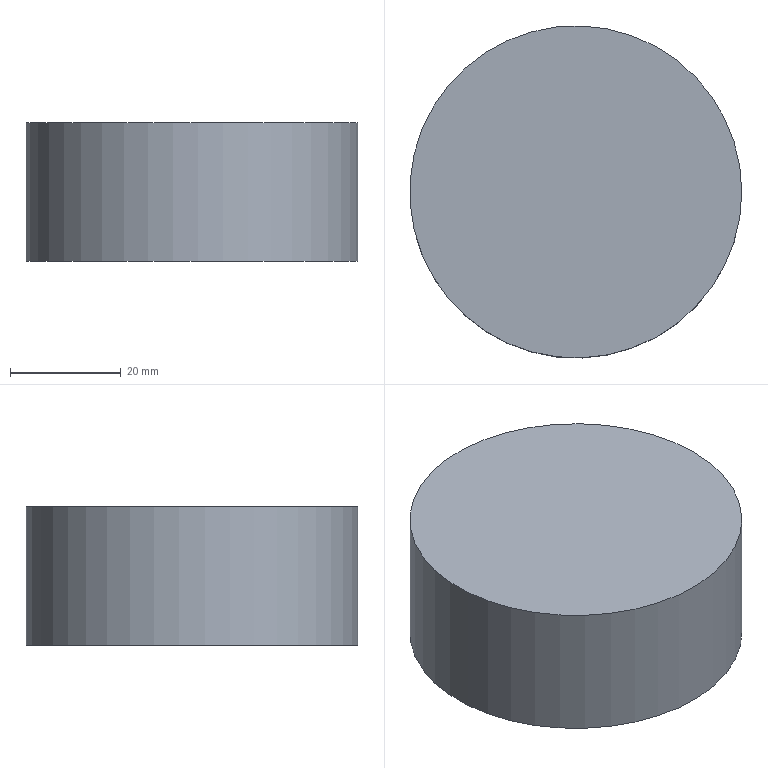Component | NX | SCREW_PLUG | 1 solid | 7 faces | box 60 x 60 x 25 mm | volume 70470 mm3 | cylinder 3 | plane 2 | cone 2 | commonest cylinder face diameters 5 x2 60 x1
STEP:
#1=CARTESIAN_POINT('',(0.,0.,0.));
#2=DIRECTION('',(0.,0.,1.));
#3=DIRECTION('',(1.,0.,0.));
#4=AXIS2_PLACEMENT_3D('',#1,#2,#3);
#5=CARTESIAN_POINT('',(24.068,1.139,38.134));
#6=VERTEX_POINT('',#5);
#7=CARTESIAN_POINT('',(-5.932,1.139,38.134));
#8=DIRECTION('',(0.,0.,-1.));
#9=DIRECTION('',(1.,0.,0.));
#10=AXIS2_PLACEMENT_3D('',#7,#8,#9);
#11=CIRCLE('',#10,30.);
#12=CARTESIAN_POINT('',(-5.932,1.139,38.134));
#13=DIRECTION('',(0.,0.,1.));
#14=DIRECTION('',(1.,0.,0.));
#15=AXIS2_PLACEMENT_3D('',#12,#13,#14);
#16=PLANE('',#15);
#17=CARTESIAN_POINT('',(30.,0.));
#18=CARTESIAN_POINT('',(30.,-51.962));
#19=CARTESIAN_POINT('',(-15.,-25.981));
#20=CARTESIAN_POINT('',(-60.,-0.));
#21=CARTESIAN_POINT('',(-15.,25.981));
#22=CARTESIAN_POINT('',(30.,51.962));
#23=CARTESIAN_POINT('',(30.,0.));
#24=(BOUNDED_CURVE()B_SPLINE_CURVE(2,(#17,#18,#19,#20,#21,#22,#23),.UNSPECIFIED.,.T.,.F.)B_SPLINE_CURVE_WITH_KNOTS((1,2,2,2,2,1),(-2.094,0.,2.094,4.189,6.283,8.378),.UNSPECIFIED.)CURVE()GEOMETRIC_REPRESENTATION_ITEM()RATIONAL_B_SPLINE_CURVE((1.,0.5,1.,0.5,1.,0.5,1.))REPRESENTATION_ITEM(''));
#25=(GEOMETRIC_REPRESENTATION_CONTEXT(2)PARAMETRIC_REPRESENTATION_CONTEXT()REPRESENTATION_CONTEXT('',''));
#26=DEFINITIONAL_REPRESENTATION('',(#24),#25);
#27=PCURVE('',#16,#26);
#28=CARTESIAN_POINT('',(-5.932,1.139,13.134));
#29=DIRECTION('',(0.,0.,1.));
#30=DIRECTION('',(1.,0.,0.));
#31=AXIS2_PLACEMENT_3D('',#28,#29,#30);
#32=CYLINDRICAL_SURFACE('',#31,30.);
#33=CARTESIAN_POINT('',(6.283,25.));
#34=DIRECTION('',(-1.,0.));
#35=VECTOR('',#34,1.);
#36=LINE('',#33,#35);
#37=(GEOMETRIC_REPRESENTATION_CONTEXT(2)PARAMETRIC_REPRESENTATION_CONTEXT()REPRESENTATION_CONTEXT('',''));
#38=DEFINITIONAL_REPRESENTATION('',(#36),#37);
#39=PCURVE('',#32,#38);
#40=SURFACE_CURVE('',#11,(#27,#39),.PCURVE_S1.);
#41=EDGE_CURVE('',#6,#6,#40,.T.);
#42=ORIENTED_EDGE('',*,*,#41,.F.);
#43=EDGE_LOOP('',(#42));
#44=FACE_BOUND('',#43,.T.);
#45=ADVANCED_FACE('',(#44),#16,.T.);
#46=CARTESIAN_POINT('',(14.068,1.139,13.134));
#47=VERTEX_POINT('',#46);
#48=CARTESIAN_POINT('',(11.568,1.139,13.134));
#49=DIRECTION('',(0.,0.,1.));
#50=DIRECTION('',(1.,0.,0.));
#51=AXIS2_PLACEMENT_3D('',#48,#49,#50);
#52=CIRCLE('',#51,2.5);
#53=CARTESIAN_POINT('',(-5.932,1.139,13.134));
#54=DIRECTION('',(0.,0.,-1.));
#55=DIRECTION('',(-1.,0.,0.));
#56=AXIS2_PLACEMENT_3D('',#53,#54,#55);
#57=PLANE('',#56);
#58=CARTESIAN_POINT('',(-20.,0.));
#59=CARTESIAN_POINT('',(-20.,4.33));
#60=CARTESIAN_POINT('',(-16.25,2.165));
#61=CARTESIAN_POINT('',(-12.5,0.));
#62=CARTESIAN_POINT('',(-16.25,-2.165));
#63=CARTESIAN_POINT('',(-20.,-4.33));
#64=CARTESIAN_POINT('',(-20.,0.));
#65=(BOUNDED_CURVE()B_SPLINE_CURVE(2,(#58,#59,#60,#61,#62,#63,#64),.UNSPECIFIED.,.T.,.F.)B_SPLINE_CURVE_WITH_KNOTS((1,2,2,2,2,1),(-2.094,0.,2.094,4.189,6.283,8.378),.UNSPECIFIED.)CURVE()GEOMETRIC_REPRESENTATION_ITEM()RATIONAL_B_SPLINE_CURVE((1.,0.5,1.,0.5,1.,0.5,1.))REPRESENTATION_ITEM(''));
#66=(GEOMETRIC_REPRESENTATION_CONTEXT(2)PARAMETRIC_REPRESENTATION_CONTEXT()REPRESENTATION_CONTEXT('',''));
#67=DEFINITIONAL_REPRESENTATION('',(#65),#66);
#68=PCURVE('',#57,#67);
#69=CARTESIAN_POINT('',(11.568,1.139,13.134));
#70=DIRECTION('',(0.,0.,1.));
#71=DIRECTION('',(1.,0.,0.));
#72=AXIS2_PLACEMENT_3D('',#69,#70,#71);
#73=CYLINDRICAL_SURFACE('',#72,2.5);
#74=CARTESIAN_POINT('',(0.,0.));
#75=DIRECTION('',(1.,0.));
#76=VECTOR('',#75,1.);
#77=LINE('',#74,#76);
#78=(GEOMETRIC_REPRESENTATION_CONTEXT(2)PARAMETRIC_REPRESENTATION_CONTEXT()REPRESENTATION_CONTEXT('',''));
#79=DEFINITIONAL_REPRESENTATION('',(#77),#78);
#80=PCURVE('',#73,#79);
#81=SURFACE_CURVE('',#52,(#68,#80),.PCURVE_S1.);
#82=EDGE_CURVE('',#47,#47,#81,.T.);
#83=ORIENTED_EDGE('',*,*,#82,.T.);
#84=EDGE_LOOP('',(#83));
#85=FACE_BOUND('',#84,.T.);
#86=CARTESIAN_POINT('',(-20.932,1.139,13.134));
#87=VERTEX_POINT('',#86);
#88=CARTESIAN_POINT('',(-23.432,1.139,13.134));
#89=DIRECTION('',(0.,0.,1.));
#90=DIRECTION('',(1.,0.,0.));
#91=AXIS2_PLACEMENT_3D('',#88,#89,#90);
#92=CIRCLE('',#91,2.5);
#93=CARTESIAN_POINT('',(15.,0.));
#94=CARTESIAN_POINT('',(15.,4.33));
#95=CARTESIAN_POINT('',(18.75,2.165));
#96=CARTESIAN_POINT('',(22.5,0.));
#97=CARTESIAN_POINT('',(18.75,-2.165));
#98=CARTESIAN_POINT('',(15.,-4.33));
#99=CARTESIAN_POINT('',(15.,0.));
#100=(BOUNDED_CURVE()B_SPLINE_CURVE(2,(#93,#94,#95,#96,#97,#98,#99),.UNSPECIFIED.,.T.,.F.)B_SPLINE_CURVE_WITH_KNOTS((1,2,2,2,2,1),(-2.094,0.,2.094,4.189,6.283,8.378),.UNSPECIFIED.)CURVE()GEOMETRIC_REPRESENTATION_ITEM()RATIONAL_B_SPLINE_CURVE((1.,0.5,1.,0.5,1.,0.5,1.))REPRESENTATION_ITEM(''));
#101=(GEOMETRIC_REPRESENTATION_CONTEXT(2)PARAMETRIC_REPRESENTATION_CONTEXT()REPRESENTATION_CONTEXT('',''));
#102=DEFINITIONAL_REPRESENTATION('',(#100),#101);
#103=PCURVE('',#57,#102);
#104=CARTESIAN_POINT('',(-23.432,1.139,13.134));
#105=DIRECTION('',(0.,0.,1.));
#106=DIRECTION('',(1.,0.,0.));
#107=AXIS2_PLACEMENT_3D('',#104,#105,#106);
#108=CYLINDRICAL_SURFACE('',#107,2.5);
#109=CARTESIAN_POINT('',(0.,0.));
#110=DIRECTION('',(1.,0.));
#111=VECTOR('',#110,1.);
#112=LINE('',#109,#111);
#113=(GEOMETRIC_REPRESENTATION_CONTEXT(2)PARAMETRIC_REPRESENTATION_CONTEXT()REPRESENTATION_CONTEXT('',''));
#114=DEFINITIONAL_REPRESENTATION('',(#112),#113);
#115=PCURVE('',#108,#114);
#116=SURFACE_CURVE('',#92,(#103,#115),.PCURVE_S1.);
#117=EDGE_CURVE('',#87,#87,#116,.T.);
#118=ORIENTED_EDGE('',*,*,#117,.T.);
#119=EDGE_LOOP('',(#118));
#120=FACE_BOUND('',#119,.T.);
#121=CARTESIAN_POINT('',(24.068,1.139,13.134));
#122=VERTEX_POINT('',#121);
#123=CARTESIAN_POINT('',(-5.932,1.139,13.134));
#124=DIRECTION('',(0.,0.,1.));
#125=DIRECTION('',(1.,0.,0.));
#126=AXIS2_PLACEMENT_3D('',#123,#124,#125);
#127=CIRCLE('',#126,30.);
#128=CARTESIAN_POINT('',(-30.,0.));
#129=CARTESIAN_POINT('',(-30.,51.962));
#130=CARTESIAN_POINT('',(15.,25.981));
#131=CARTESIAN_POINT('',(60.,0.));
#132=CARTESIAN_POINT('',(15.,-25.981));
#133=CARTESIAN_POINT('',(-30.,-51.962));
#134=CARTESIAN_POINT('',(-30.,0.));
#135=(BOUNDED_CURVE()B_SPLINE_CURVE(2,(#128,#129,#130,#131,#132,#133,#134),.UNSPECIFIED.,.T.,.F.)B_SPLINE_CURVE_WITH_KNOTS((1,2,2,2,2,1),(-2.094,0.,2.094,4.189,6.283,8.378),.UNSPECIFIED.)CURVE()GEOMETRIC_REPRESENTATION_ITEM()RATIONAL_B_SPLINE_CURVE((1.,0.5,1.,0.5,1.,0.5,1.))REPRESENTATION_ITEM(''));
#136=(GEOMETRIC_REPRESENTATION_CONTEXT(2)PARAMETRIC_REPRESENTATION_CONTEXT()REPRESENTATION_CONTEXT('',''));
#137=DEFINITIONAL_REPRESENTATION('',(#135),#136);
#138=PCURVE('',#57,#137);
#139=CARTESIAN_POINT('',(0.,0.));
#140=DIRECTION('',(1.,0.));
#141=VECTOR('',#140,1.);
#142=LINE('',#139,#141);
#143=(GEOMETRIC_REPRESENTATION_CONTEXT(2)PARAMETRIC_REPRESENTATION_CONTEXT()REPRESENTATION_CONTEXT('',''));
#144=DEFINITIONAL_REPRESENTATION('',(#142),#143);
#145=PCURVE('',#32,#144);
#146=SURFACE_CURVE('',#127,(#138,#145),.PCURVE_S1.);
#147=EDGE_CURVE('',#122,#122,#146,.T.);
#148=ORIENTED_EDGE('',*,*,#147,.F.);
#149=EDGE_LOOP('',(#148));
#150=FACE_BOUND('',#149,.T.);
#151=ADVANCED_FACE('',(#85,#120,#150),#57,.T.);
#152=ORIENTED_EDGE('',*,*,#41,.T.);
#153=CARTESIAN_POINT('',(24.068,1.139,13.134));
#154=CARTESIAN_POINT('',(24.068,1.139,38.134));
#155=B_SPLINE_CURVE_WITH_KNOTS('',1,(#153,#154),.UNSPECIFIED.,.F.,.F.,(2,2),(0.,25.),.PIECEWISE_BEZIER_KNOTS.);
#156=CARTESIAN_POINT('',(0.,0.));
#157=DIRECTION('',(0.,1.));
#158=VECTOR('',#157,1.);
#159=LINE('',#156,#158);
#160=(GEOMETRIC_REPRESENTATION_CONTEXT(2)PARAMETRIC_REPRESENTATION_CONTEXT()REPRESENTATION_CONTEXT('',''));
#161=DEFINITIONAL_REPRESENTATION('',(#159),#160);
#162=PCURVE('',#32,#161);
#163=CARTESIAN_POINT('',(6.283,0.));
#164=DIRECTION('',(0.,1.));
#165=VECTOR('',#164,1.);
#166=LINE('',#163,#165);
#167=(GEOMETRIC_REPRESENTATION_CONTEXT(2)PARAMETRIC_REPRESENTATION_CONTEXT()REPRESENTATION_CONTEXT('',''));
#168=DEFINITIONAL_REPRESENTATION('',(#166),#167);
#169=PCURVE('',#32,#168);
#170=SEAM_CURVE('',#155,(#162,#169),.PCURVE_S1.);
#171=EDGE_CURVE('',#122,#6,#170,.T.);
#172=ORIENTED_EDGE('',*,*,#171,.F.);
#173=ORIENTED_EDGE('',*,*,#147,.T.);
#174=ORIENTED_EDGE('',*,*,#171,.T.);
#175=EDGE_LOOP('',(#152,#172,#173,#174));
#176=FACE_BOUND('',#175,.T.);
#177=ADVANCED_FACE('',(#176),#32,.T.);
#178=CARTESIAN_POINT('',(-25.932,1.139,18.134));
#179=VERTEX_POINT('',#178);
#180=CARTESIAN_POINT('',(-20.932,1.139,18.134));
#181=VERTEX_POINT('',#180);
#182=CARTESIAN_POINT('',(-23.432,1.139,18.134));
#183=DIRECTION('',(0.,0.,-1.));
#184=DIRECTION('',(1.,0.,0.));
#185=AXIS2_PLACEMENT_3D('',#182,#183,#184);
#186=CIRCLE('',#185,2.5);
#187=CARTESIAN_POINT('',(-23.432,1.139,18.134));
#188=DIRECTION('',(0.,0.,-1.));
#189=DIRECTION('',(-1.,0.,0.));
#190=AXIS2_PLACEMENT_3D('',#187,#188,#189);
#191=CONICAL_SURFACE('',#190,2.5,1.03);
#192=CARTESIAN_POINT('',(-3.142,0.));
#193=DIRECTION('',(1.,0.));
#194=VECTOR('',#193,1.);
#195=LINE('',#192,#194);
#196=(GEOMETRIC_REPRESENTATION_CONTEXT(2)PARAMETRIC_REPRESENTATION_CONTEXT()REPRESENTATION_CONTEXT('',''));
#197=DEFINITIONAL_REPRESENTATION('',(#195),#196);
#198=PCURVE('',#191,#197);
#199=CARTESIAN_POINT('',(6.283,5.));
#200=DIRECTION('',(-1.,0.));
#201=VECTOR('',#200,1.);
#202=LINE('',#199,#201);
#203=(GEOMETRIC_REPRESENTATION_CONTEXT(2)PARAMETRIC_REPRESENTATION_CONTEXT()REPRESENTATION_CONTEXT('',''));
#204=DEFINITIONAL_REPRESENTATION('',(#202),#203);
#205=PCURVE('',#108,#204);
#206=SURFACE_CURVE('',#186,(#198,#205),.PCURVE_S1.);
#207=EDGE_CURVE('',#179,#181,#206,.T.);
#208=ORIENTED_EDGE('',*,*,#207,.F.);
#209=CARTESIAN_POINT('',(-23.432,1.139,19.636));
#210=VERTEX_POINT('',#209);
#211=CARTESIAN_POINT('',(-23.432,1.139,19.636));
#212=CARTESIAN_POINT('',(-25.932,1.139,18.134));
#213=B_SPLINE_CURVE_WITH_KNOTS('',1,(#211,#212),.UNSPECIFIED.,.F.,.F.,(2,2),(-2.917,0.),.PIECEWISE_BEZIER_KNOTS.);
#214=CARTESIAN_POINT('',(0.,0.));
#215=DIRECTION('',(0.,1.));
#216=VECTOR('',#215,1.);
#217=LINE('',#214,#216);
#218=(GEOMETRIC_REPRESENTATION_CONTEXT(2)PARAMETRIC_REPRESENTATION_CONTEXT()REPRESENTATION_CONTEXT('',''));
#219=DEFINITIONAL_REPRESENTATION('',(#217),#218);
#220=PCURVE('',#191,#219);
#221=CARTESIAN_POINT('',(6.283,0.));
#222=DIRECTION('',(0.,1.));
#223=VECTOR('',#222,1.);
#224=LINE('',#221,#223);
#225=(GEOMETRIC_REPRESENTATION_CONTEXT(2)PARAMETRIC_REPRESENTATION_CONTEXT()REPRESENTATION_CONTEXT('',''));
#226=DEFINITIONAL_REPRESENTATION('',(#224),#225);
#227=PCURVE('',#191,#226);
#228=SEAM_CURVE('',#213,(#220,#227),.PCURVE_S1.);
#229=EDGE_CURVE('',#210,#179,#228,.T.);
#230=ORIENTED_EDGE('',*,*,#229,.F.);
#231=ORIENTED_EDGE('',*,*,#229,.T.);
#232=CARTESIAN_POINT('',(-23.432,1.139,18.134));
#233=DIRECTION('',(0.,0.,-1.));
#234=DIRECTION('',(1.,0.,0.));
#235=AXIS2_PLACEMENT_3D('',#232,#233,#234);
#236=CIRCLE('',#235,2.5);
#237=CARTESIAN_POINT('',(3.142,0.));
#238=DIRECTION('',(1.,0.));
#239=VECTOR('',#238,1.);
#240=LINE('',#237,#239);
#241=(GEOMETRIC_REPRESENTATION_CONTEXT(2)PARAMETRIC_REPRESENTATION_CONTEXT()REPRESENTATION_CONTEXT('',''));
#242=DEFINITIONAL_REPRESENTATION('',(#240),#241);
#243=PCURVE('',#191,#242);
#244=CARTESIAN_POINT('',(6.283,5.));
#245=DIRECTION('',(-1.,0.));
#246=VECTOR('',#245,1.);
#247=LINE('',#244,#246);
#248=(GEOMETRIC_REPRESENTATION_CONTEXT(2)PARAMETRIC_REPRESENTATION_CONTEXT()REPRESENTATION_CONTEXT('',''));
#249=DEFINITIONAL_REPRESENTATION('',(#247),#248);
#250=PCURVE('',#108,#249);
#251=SURFACE_CURVE('',#236,(#243,#250),.PCURVE_S1.);
#252=EDGE_CURVE('',#181,#179,#251,.T.);
#253=ORIENTED_EDGE('',*,*,#252,.F.);
#254=EDGE_LOOP('',(#208,#230,#231,#253));
#255=FACE_BOUND('',#254,.F.);
#256=ADVANCED_FACE('',(#255),#191,.F.);
#257=ORIENTED_EDGE('',*,*,#207,.T.);
#258=CARTESIAN_POINT('',(-20.932,1.139,13.134));
#259=CARTESIAN_POINT('',(-20.932,1.139,18.134));
#260=B_SPLINE_CURVE_WITH_KNOTS('',1,(#258,#259),.UNSPECIFIED.,.F.,.F.,(2,2),(0.,5.),.PIECEWISE_BEZIER_KNOTS.);
#261=CARTESIAN_POINT('',(0.,0.));
#262=DIRECTION('',(0.,1.));
#263=VECTOR('',#262,1.);
#264=LINE('',#261,#263);
#265=(GEOMETRIC_REPRESENTATION_CONTEXT(2)PARAMETRIC_REPRESENTATION_CONTEXT()REPRESENTATION_CONTEXT('',''));
#266=DEFINITIONAL_REPRESENTATION('',(#264),#265);
#267=PCURVE('',#108,#266);
#268=CARTESIAN_POINT('',(6.283,0.));
#269=DIRECTION('',(0.,1.));
#270=VECTOR('',#269,1.);
#271=LINE('',#268,#270);
#272=(GEOMETRIC_REPRESENTATION_CONTEXT(2)PARAMETRIC_REPRESENTATION_CONTEXT()REPRESENTATION_CONTEXT('',''));
#273=DEFINITIONAL_REPRESENTATION('',(#271),#272);
#274=PCURVE('',#108,#273);
#275=SEAM_CURVE('',#260,(#267,#274),.PCURVE_S1.);
#276=EDGE_CURVE('',#87,#181,#275,.T.);
#277=ORIENTED_EDGE('',*,*,#276,.F.);
#278=ORIENTED_EDGE('',*,*,#117,.T.);
#279=ORIENTED_EDGE('',*,*,#276,.T.);
#280=ORIENTED_EDGE('',*,*,#252,.T.);
#281=EDGE_LOOP('',(#257,#277,#278,#279,#280));
#282=FACE_BOUND('',#281,.F.);
#283=ADVANCED_FACE('',(#282),#108,.F.);
#284=CARTESIAN_POINT('',(9.068,1.139,18.134));
#285=VERTEX_POINT('',#284);
#286=CARTESIAN_POINT('',(14.068,1.139,18.134));
#287=VERTEX_POINT('',#286);
#288=CARTESIAN_POINT('',(11.568,1.139,18.134));
#289=DIRECTION('',(0.,0.,-1.));
#290=DIRECTION('',(1.,0.,0.));
#291=AXIS2_PLACEMENT_3D('',#288,#289,#290);
#292=CIRCLE('',#291,2.5);
#293=CARTESIAN_POINT('',(11.568,1.139,18.134));
#294=DIRECTION('',(0.,0.,-1.));
#295=DIRECTION('',(-1.,0.,0.));
#296=AXIS2_PLACEMENT_3D('',#293,#294,#295);
#297=CONICAL_SURFACE('',#296,2.5,1.03);
#298=CARTESIAN_POINT('',(-3.142,0.));
#299=DIRECTION('',(1.,0.));
#300=VECTOR('',#299,1.);
#301=LINE('',#298,#300);
#302=(GEOMETRIC_REPRESENTATION_CONTEXT(2)PARAMETRIC_REPRESENTATION_CONTEXT()REPRESENTATION_CONTEXT('',''));
#303=DEFINITIONAL_REPRESENTATION('',(#301),#302);
#304=PCURVE('',#297,#303);
#305=CARTESIAN_POINT('',(6.283,5.));
#306=DIRECTION('',(-1.,0.));
#307=VECTOR('',#306,1.);
#308=LINE('',#305,#307);
#309=(GEOMETRIC_REPRESENTATION_CONTEXT(2)PARAMETRIC_REPRESENTATION_CONTEXT()REPRESENTATION_CONTEXT('',''));
#310=DEFINITIONAL_REPRESENTATION('',(#308),#309);
#311=PCURVE('',#73,#310);
#312=SURFACE_CURVE('',#292,(#304,#311),.PCURVE_S1.);
#313=EDGE_CURVE('',#285,#287,#312,.T.);
#314=ORIENTED_EDGE('',*,*,#313,.F.);
#315=CARTESIAN_POINT('',(11.568,1.139,19.636));
#316=VERTEX_POINT('',#315);
#317=CARTESIAN_POINT('',(11.568,1.139,19.636));
#318=CARTESIAN_POINT('',(9.068,1.139,18.134));
#319=B_SPLINE_CURVE_WITH_KNOTS('',1,(#317,#318),.UNSPECIFIED.,.F.,.F.,(2,2),(-2.917,0.),.PIECEWISE_BEZIER_KNOTS.);
#320=CARTESIAN_POINT('',(0.,0.));
#321=DIRECTION('',(0.,1.));
#322=VECTOR('',#321,1.);
#323=LINE('',#320,#322);
#324=(GEOMETRIC_REPRESENTATION_CONTEXT(2)PARAMETRIC_REPRESENTATION_CONTEXT()REPRESENTATION_CONTEXT('',''));
#325=DEFINITIONAL_REPRESENTATION('',(#323),#324);
#326=PCURVE('',#297,#325);
#327=CARTESIAN_POINT('',(6.283,0.));
#328=DIRECTION('',(0.,1.));
#329=VECTOR('',#328,1.);
#330=LINE('',#327,#329);
#331=(GEOMETRIC_REPRESENTATION_CONTEXT(2)PARAMETRIC_REPRESENTATION_CONTEXT()REPRESENTATION_CONTEXT('',''));
#332=DEFINITIONAL_REPRESENTATION('',(#330),#331);
#333=PCURVE('',#297,#332);
#334=SEAM_CURVE('',#319,(#326,#333),.PCURVE_S1.);
#335=EDGE_CURVE('',#316,#285,#334,.T.);
#336=ORIENTED_EDGE('',*,*,#335,.F.);
#337=ORIENTED_EDGE('',*,*,#335,.T.);
#338=CARTESIAN_POINT('',(11.568,1.139,18.134));
#339=DIRECTION('',(0.,0.,-1.));
#340=DIRECTION('',(1.,0.,0.));
#341=AXIS2_PLACEMENT_3D('',#338,#339,#340);
#342=CIRCLE('',#341,2.5);
#343=CARTESIAN_POINT('',(3.142,0.));
#344=DIRECTION('',(1.,0.));
#345=VECTOR('',#344,1.);
#346=LINE('',#343,#345);
#347=(GEOMETRIC_REPRESENTATION_CONTEXT(2)PARAMETRIC_REPRESENTATION_CONTEXT()REPRESENTATION_CONTEXT('',''));
#348=DEFINITIONAL_REPRESENTATION('',(#346),#347);
#349=PCURVE('',#297,#348);
#350=CARTESIAN_POINT('',(6.283,5.));
#351=DIRECTION('',(-1.,0.));
#352=VECTOR('',#351,1.);
#353=LINE('',#350,#352);
#354=(GEOMETRIC_REPRESENTATION_CONTEXT(2)PARAMETRIC_REPRESENTATION_CONTEXT()REPRESENTATION_CONTEXT('',''));
#355=DEFINITIONAL_REPRESENTATION('',(#353),#354);
#356=PCURVE('',#73,#355);
#357=SURFACE_CURVE('',#342,(#349,#356),.PCURVE_S1.);
#358=EDGE_CURVE('',#287,#285,#357,.T.);
#359=ORIENTED_EDGE('',*,*,#358,.F.);
#360=EDGE_LOOP('',(#314,#336,#337,#359));
#361=FACE_BOUND('',#360,.F.);
#362=ADVANCED_FACE('',(#361),#297,.F.);
#363=ORIENTED_EDGE('',*,*,#313,.T.);
#364=CARTESIAN_POINT('',(14.068,1.139,13.134));
#365=CARTESIAN_POINT('',(14.068,1.139,18.134));
#366=B_SPLINE_CURVE_WITH_KNOTS('',1,(#364,#365),.UNSPECIFIED.,.F.,.F.,(2,2),(0.,5.),.PIECEWISE_BEZIER_KNOTS.);
#367=CARTESIAN_POINT('',(0.,0.));
#368=DIRECTION('',(0.,1.));
#369=VECTOR('',#368,1.);
#370=LINE('',#367,#369);
#371=(GEOMETRIC_REPRESENTATION_CONTEXT(2)PARAMETRIC_REPRESENTATION_CONTEXT()REPRESENTATION_CONTEXT('',''));
#372=DEFINITIONAL_REPRESENTATION('',(#370),#371);
#373=PCURVE('',#73,#372);
#374=CARTESIAN_POINT('',(6.283,0.));
#375=DIRECTION('',(0.,1.));
#376=VECTOR('',#375,1.);
#377=LINE('',#374,#376);
#378=(GEOMETRIC_REPRESENTATION_CONTEXT(2)PARAMETRIC_REPRESENTATION_CONTEXT()REPRESENTATION_CONTEXT('',''));
#379=DEFINITIONAL_REPRESENTATION('',(#377),#378);
#380=PCURVE('',#73,#379);
#381=SEAM_CURVE('',#366,(#373,#380),.PCURVE_S1.);
#382=EDGE_CURVE('',#47,#287,#381,.T.);
#383=ORIENTED_EDGE('',*,*,#382,.F.);
#384=ORIENTED_EDGE('',*,*,#82,.T.);
#385=ORIENTED_EDGE('',*,*,#382,.T.);
#386=ORIENTED_EDGE('',*,*,#358,.T.);
#387=EDGE_LOOP('',(#363,#383,#384,#385,#386));
#388=FACE_BOUND('',#387,.F.);
#389=ADVANCED_FACE('',(#388),#73,.F.);
#390=CLOSED_SHELL('',(#45,#151,#177,#256,#283,#362,#389));
#391=MANIFOLD_SOLID_BREP('',#390);
#392=(LENGTH_UNIT()NAMED_UNIT(*)SI_UNIT(.MILLI.,.METRE.));
#393=UNCERTAINTY_MEASURE_WITH_UNIT(LENGTH_MEASURE(0.00001),#392,'','');
#394=(NAMED_UNIT(*)PLANE_ANGLE_UNIT()SI_UNIT($,.RADIAN.));
#395=(NAMED_UNIT(*)SI_UNIT($,.STERADIAN.)SOLID_ANGLE_UNIT());
#396=(GEOMETRIC_REPRESENTATION_CONTEXT(3)GLOBAL_UNCERTAINTY_ASSIGNED_CONTEXT((#393))GLOBAL_UNIT_ASSIGNED_CONTEXT((#392,#394,#395))REPRESENTATION_CONTEXT('',''));
#397=ADVANCED_BREP_SHAPE_REPRESENTATION('',(#4,#391),#396);